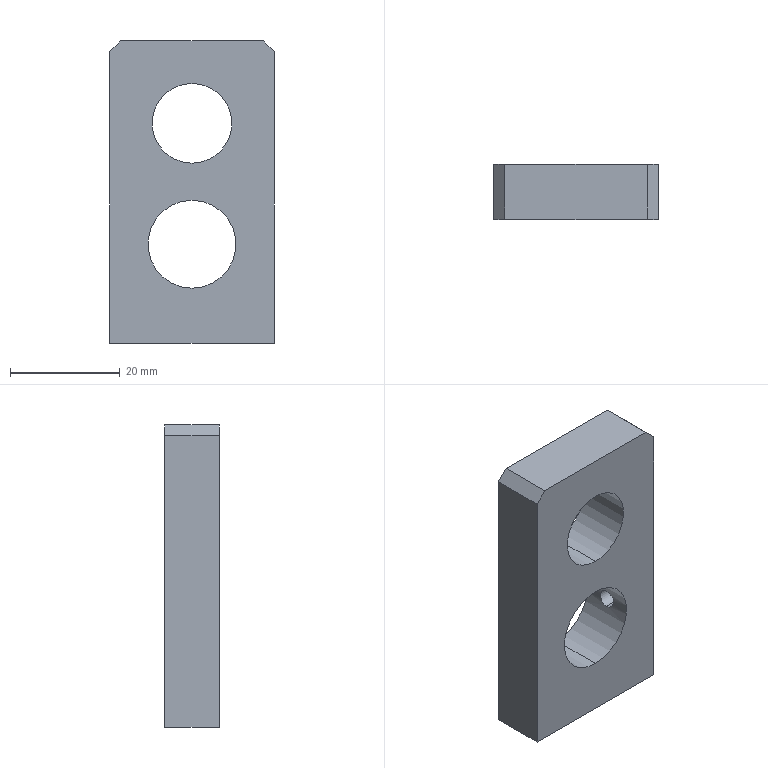Component | SolidWorks | GbgbMagnetSleeveSeatF8-4 | 1 solid | 22 faces | box 30 x 10 x 55 mm | volume 12559 mm3 | cylinder 10 | plane 8 | cone 4 | commonest cylinder face diameters 3.3 x6 14.5 x2 16 x2
build123d program:
from build123d import *

# Parameters (mm, degrees)
SKETCH1_W              = 30
SKETCH1_H              = 55
BOSS_EXTRUDE1_DEPTH    = 5
SKETCH2_R              = 6
CUT_EXTRUDE1_DEPTH     = 33.882
M4_TAPPED_HOLE2_D      = 3.3
M4_TAPPED_HOLE2_DEPTH  = 10.1
M4_TAPPED_HOLE2_TIP    = 0.9914
SKETCH12_R             = 8
CUT_EXTRUDE2_DEPTH     = 12
M16X1_5_TAPPED_HOLE1_D = 14.5
M4_TAPPED_HOLE3_D      = 3.3
M4_TAPPED_HOLE3_DEPTH  = 10.1
M4_TAPPED_HOLE3_TIP    = 0.9914
CHAMFER1_SIZE          = 2


with BuildPart() as part:
    # Sketch1 → Boss-Extrude1 (new, symmetric)
    with BuildSketch(Plane(origin=(0, 0, 0), x_dir=(1, 0, 0), z_dir=(0, 1, 0))):
        Rectangle(SKETCH1_W, SKETCH1_H)
    extrude(amount=BOSS_EXTRUDE1_DEPTH, both=True)

    # Sketch2 → Cut-Extrude1 (cut, through all)
    with BuildSketch(Plane(origin=(0, 5, 0), x_dir=(1, 0, 0), z_dir=(0, 1, 0))):
        with Locations(Location((0, -12.5, 0), (0, 0, 270))):
            Circle(SKETCH2_R)
    extrude(amount=-CUT_EXTRUDE1_DEPTH, mode=Mode.SUBTRACT)

    # M4 Tapped Hole2
    with Locations(Plane(origin=(2.316, -9.359, -27.5), x_dir=(1, 0, 0), z_dir=(0, 0, -1))):
        with Locations((7.684, -9.359), (-12.316, -9.359)):
            Hole(M4_TAPPED_HOLE2_D / 2, depth=M4_TAPPED_HOLE2_DEPTH)
            with Locations((0, 0, -(M4_TAPPED_HOLE2_DEPTH + M4_TAPPED_HOLE2_TIP / 2))):  # 118° drill point
                Cone(0, M4_TAPPED_HOLE2_D / 2, M4_TAPPED_HOLE2_TIP, mode=Mode.SUBTRACT)

    # Sketch12 → Cut-Extrude2 (cut)
    with BuildSketch(Plane(origin=(0, 5, 0), x_dir=(1, 0, 0), z_dir=(0, 1, 0))):
        with Locations(Location((0, 9.5, 0), (0, 0, 270))):
            Circle(SKETCH12_R)
    extrude(amount=-CUT_EXTRUDE2_DEPTH, mode=Mode.SUBTRACT)

    # M16x1.5 Tapped Hole1 (through all)
    with Locations(Plane(origin=(0, 5, 0), x_dir=(1, 0, 0), z_dir=(0, 1, 0))):
        with Locations((0, -12.5)):
            Hole(M16X1_5_TAPPED_HOLE1_D / 2)

    # M4 Tapped Hole3
    with Locations(Plane(origin=(15, 0, 0), x_dir=(0, 0, -1), z_dir=(1, 0, 0))):
        with Locations((9.5, 0)):
            Hole(M4_TAPPED_HOLE3_D / 2, depth=M4_TAPPED_HOLE3_DEPTH)
            with Locations((0, 0, -(M4_TAPPED_HOLE3_DEPTH + M4_TAPPED_HOLE3_TIP / 2))):  # 118° drill point
                Cone(0, M4_TAPPED_HOLE3_D / 2, M4_TAPPED_HOLE3_TIP, mode=Mode.SUBTRACT)

    # Chamfer1
    chamfer1_edges = [part.edges().sort_by_distance(p)[0] for p in [
        (15, 0, 27.5),
        (-15, 0, 27.5),
    ]]
    chamfer(chamfer1_edges, length=CHAMFER1_SIZE)


solid = part.part

# Placed as in the assembly
solid = solid.moved(Location((80.446, 494.94, 417.732), (0, 0, 0)))
STEP:
#1=CARTESIAN_POINT('',(3.475,19.486,16.137));
#2=VERTEX_POINT('',#1);
#3=CARTESIAN_POINT('',(3.475,19.486,16.007));
#4=VERTEX_POINT('',#3);
#5=CARTESIAN_POINT('',(3.475,19.486,16.137));
#6=CARTESIAN_POINT('',(3.475,19.477,16.137));
#7=CARTESIAN_POINT('',(3.476,19.469,16.135));
#8=CARTESIAN_POINT('',(3.477,19.457,16.13));
#9=CARTESIAN_POINT('',(3.477,19.453,16.128));
#10=CARTESIAN_POINT('',(3.478,19.446,16.124));
#11=CARTESIAN_POINT('',(3.478,19.443,16.121));
#12=CARTESIAN_POINT('',(3.479,19.437,16.115));
#13=CARTESIAN_POINT('',(3.48,19.434,16.112));
#14=CARTESIAN_POINT('',(3.48,19.429,16.105));
#15=CARTESIAN_POINT('',(3.481,19.427,16.101));
#16=CARTESIAN_POINT('',(3.482,19.423,16.089));
#17=CARTESIAN_POINT('',(3.482,19.421,16.081));
#18=CARTESIAN_POINT('',(3.482,19.421,16.068));
#19=CARTESIAN_POINT('',(3.482,19.421,16.064));
#20=CARTESIAN_POINT('',(3.482,19.423,16.055));
#21=CARTESIAN_POINT('',(3.481,19.424,16.051));
#22=CARTESIAN_POINT('',(3.481,19.427,16.043));
#23=CARTESIAN_POINT('',(3.48,19.429,16.04));
#24=CARTESIAN_POINT('',(3.48,19.434,16.033));
#25=CARTESIAN_POINT('',(3.479,19.437,16.029));
#26=CARTESIAN_POINT('',(3.478,19.446,16.02));
#27=CARTESIAN_POINT('',(3.477,19.453,16.015));
#28=CARTESIAN_POINT('',(3.476,19.465,16.011));
#29=CARTESIAN_POINT('',(3.476,19.469,16.009));
#30=CARTESIAN_POINT('',(3.475,19.477,16.008));
#31=CARTESIAN_POINT('',(3.475,19.482,16.007));
#32=CARTESIAN_POINT('',(3.475,19.486,16.007));
#33=B_SPLINE_CURVE_WITH_KNOTS('',3,(#5,#6,#7,#8,#9,#10,#11,#12,#13,#14,#15,#16,#17,#18,#19,#20,#21,#22,#23,#24,#25,#26,#27,#28,#29,#30,#31,#32),.UNSPECIFIED.,.F.,.F.,(4,2,2,2,2,2,2,2,2,2,2,2,2,4),(0.005173,0.005819,0.006142,0.006465,0.006789,0.007112,0.007758,0.008081,0.008405,0.008728,0.009051,0.009697,0.01002,0.01034),.UNSPECIFIED.);
#34=EDGE_CURVE('',#2,#4,#33,.T.);
#35=ORIENTED_EDGE('',*,*,#34,.F.);
#36=CARTESIAN_POINT('',(3.758,19.486,16.137));
#37=VERTEX_POINT('',#36);
#38=CARTESIAN_POINT('',(3.758,19.486,16.137));
#39=DIRECTION('',(1.,0.,-0.));
#40=VECTOR('',#39,39.37);
#41=LINE('',#38,#40);
#42=EDGE_CURVE('',#2,#37,#41,.T.);
#43=ORIENTED_EDGE('',*,*,#42,.T.);
#44=CARTESIAN_POINT('',(3.758,19.486,16.007));
#45=VERTEX_POINT('',#44);
#46=CARTESIAN_POINT('',(3.758,19.486,16.072));
#47=DIRECTION('',(1.,0.,-0.));
#48=DIRECTION('',(0.,0.,-1.));
#49=AXIS2_PLACEMENT_3D('',#46,#47,#48);
#50=CIRCLE('',#49,0.06496);
#51=EDGE_CURVE('',#37,#45,#50,.T.);
#52=ORIENTED_EDGE('',*,*,#51,.T.);
#53=CARTESIAN_POINT('',(3.758,19.486,16.007));
#54=DIRECTION('',(1.,0.,-0.));
#55=VECTOR('',#54,39.37);
#56=LINE('',#53,#55);
#57=EDGE_CURVE('',#4,#45,#56,.T.);
#58=ORIENTED_EDGE('',*,*,#57,.F.);
#59=EDGE_LOOP('',(#35,#43,#52,#58));
#60=FACE_OUTER_BOUND('',#59,.T.);
#61=CARTESIAN_POINT('',(3.758,19.486,16.072));
#62=DIRECTION('',(1.,0.,-0.));
#63=DIRECTION('',(0.,0.,-1.));
#64=AXIS2_PLACEMENT_3D('',#61,#62,#63);
#65=CYLINDRICAL_SURFACE('',#64,0.06496);
#66=ADVANCED_FACE('',(#60),#65,.F.);
#67=CARTESIAN_POINT('',(3.167,19.289,16.653));
#68=VERTEX_POINT('',#67);
#69=CARTESIAN_POINT('',(3.167,19.289,17.224));
#70=VERTEX_POINT('',#69);
#71=CARTESIAN_POINT('',(3.167,19.289,16.938));
#72=DIRECTION('',(0.,1.,0.));
#73=DIRECTION('',(0.,0.,1.));
#74=AXIS2_PLACEMENT_3D('',#71,#72,#73);
#75=CIRCLE('',#74,0.2854);
#76=EDGE_CURVE('',#68,#70,#75,.T.);
#77=ORIENTED_EDGE('',*,*,#76,.F.);
#78=CARTESIAN_POINT('',(3.167,19.683,16.653));
#79=VERTEX_POINT('',#78);
#80=CARTESIAN_POINT('',(3.167,19.683,16.653));
#81=DIRECTION('',(0.,1.,0.));
#82=VECTOR('',#81,39.37);
#83=LINE('',#80,#82);
#84=EDGE_CURVE('',#68,#79,#83,.T.);
#85=ORIENTED_EDGE('',*,*,#84,.T.);
#86=CARTESIAN_POINT('',(3.167,19.683,17.224));
#87=VERTEX_POINT('',#86);
#88=CARTESIAN_POINT('',(3.167,19.683,16.938));
#89=DIRECTION('',(0.,1.,0.));
#90=DIRECTION('',(0.,0.,1.));
#91=AXIS2_PLACEMENT_3D('',#88,#89,#90);
#92=CIRCLE('',#91,0.2854);
#93=EDGE_CURVE('',#79,#87,#92,.T.);
#94=ORIENTED_EDGE('',*,*,#93,.T.);
#95=CARTESIAN_POINT('',(3.167,19.683,17.224));
#96=DIRECTION('',(0.,1.,0.));
#97=VECTOR('',#96,39.37);
#98=LINE('',#95,#97);
#99=EDGE_CURVE('',#70,#87,#98,.T.);
#100=ORIENTED_EDGE('',*,*,#99,.F.);
#101=EDGE_LOOP('',(#77,#85,#94,#100));
#102=FACE_OUTER_BOUND('',#101,.T.);
#103=CARTESIAN_POINT('',(3.167,19.683,16.938));
#104=DIRECTION('',(0.,1.,0.));
#105=DIRECTION('',(0.,0.,1.));
#106=AXIS2_PLACEMENT_3D('',#103,#104,#105);
#107=CYLINDRICAL_SURFACE('',#106,0.2854);
#108=ADVANCED_FACE('',(#102),#107,.F.);
#109=CARTESIAN_POINT('',(3.167,19.289,15.757));
#110=VERTEX_POINT('',#109);
#111=CARTESIAN_POINT('',(3.167,19.289,16.387));
#112=VERTEX_POINT('',#111);
#113=CARTESIAN_POINT('',(3.167,19.289,16.072));
#114=DIRECTION('',(0.,1.,0.));
#115=DIRECTION('',(0.,0.,1.));
#116=AXIS2_PLACEMENT_3D('',#113,#114,#115);
#117=CIRCLE('',#116,0.315);
#118=EDGE_CURVE('',#110,#112,#117,.T.);
#119=ORIENTED_EDGE('',*,*,#118,.F.);
#120=CARTESIAN_POINT('',(3.167,19.683,15.757));
#121=VERTEX_POINT('',#120);
#122=CARTESIAN_POINT('',(3.167,19.21,15.757));
#123=DIRECTION('',(0.,1.,0.));
#124=VECTOR('',#123,39.37);
#125=LINE('',#122,#124);
#126=EDGE_CURVE('',#110,#121,#125,.T.);
#127=ORIENTED_EDGE('',*,*,#126,.T.);
#128=CARTESIAN_POINT('',(3.167,19.683,16.387));
#129=VERTEX_POINT('',#128);
#130=CARTESIAN_POINT('',(3.167,19.683,16.072));
#131=DIRECTION('',(0.,1.,0.));
#132=DIRECTION('',(0.,0.,1.));
#133=AXIS2_PLACEMENT_3D('',#130,#131,#132);
#134=CIRCLE('',#133,0.315);
#135=EDGE_CURVE('',#121,#129,#134,.T.);
#136=ORIENTED_EDGE('',*,*,#135,.T.);
#137=CARTESIAN_POINT('',(3.167,19.21,16.387));
#138=DIRECTION('',(0.,1.,0.));
#139=VECTOR('',#138,39.37);
#140=LINE('',#137,#139);
#141=EDGE_CURVE('',#112,#129,#140,.T.);
#142=ORIENTED_EDGE('',*,*,#141,.F.);
#143=EDGE_LOOP('',(#119,#127,#136,#142));
#144=FACE_OUTER_BOUND('',#143,.T.);
#145=CARTESIAN_POINT('',(3.167,19.21,16.072));
#146=DIRECTION('',(0.,1.,0.));
#147=DIRECTION('',(0.,0.,1.));
#148=AXIS2_PLACEMENT_3D('',#145,#146,#147);
#149=CYLINDRICAL_SURFACE('',#148,0.315);
#150=ADVANCED_FACE('',(#144),#149,.F.);
#151=CARTESIAN_POINT('',(3.626,19.486,15.761));
#152=VERTEX_POINT('',#151);
#153=CARTESIAN_POINT('',(3.496,19.486,15.761));
#154=VERTEX_POINT('',#153);
#155=CARTESIAN_POINT('',(3.561,19.486,15.761));
#156=DIRECTION('',(0.,0.,-1.));
#157=DIRECTION('',(-1.,0.,0.));
#158=AXIS2_PLACEMENT_3D('',#155,#156,#157);
#159=CIRCLE('',#158,0.06496);
#160=EDGE_CURVE('',#152,#154,#159,.T.);
#161=ORIENTED_EDGE('',*,*,#160,.F.);
#162=CARTESIAN_POINT('',(3.626,19.486,15.363));
#163=VERTEX_POINT('',#162);
#164=CARTESIAN_POINT('',(3.626,19.486,15.363));
#165=DIRECTION('',(0.,0.,-1.));
#166=VECTOR('',#165,39.37);
#167=LINE('',#164,#166);
#168=EDGE_CURVE('',#152,#163,#167,.T.);
#169=ORIENTED_EDGE('',*,*,#168,.T.);
#170=CARTESIAN_POINT('',(3.496,19.486,15.363));
#171=VERTEX_POINT('',#170);
#172=CARTESIAN_POINT('',(3.561,19.486,15.363));
#173=DIRECTION('',(0.,0.,-1.));
#174=DIRECTION('',(-1.,0.,0.));
#175=AXIS2_PLACEMENT_3D('',#172,#173,#174);
#176=CIRCLE('',#175,0.06496);
#177=EDGE_CURVE('',#163,#171,#176,.T.);
#178=ORIENTED_EDGE('',*,*,#177,.T.);
#179=CARTESIAN_POINT('',(3.496,19.486,15.363));
#180=DIRECTION('',(0.,0.,-1.));
#181=VECTOR('',#180,39.37);
#182=LINE('',#179,#181);
#183=EDGE_CURVE('',#154,#171,#182,.T.);
#184=ORIENTED_EDGE('',*,*,#183,.F.);
#185=EDGE_LOOP('',(#161,#169,#178,#184));
#186=FACE_OUTER_BOUND('',#185,.T.);
#187=CARTESIAN_POINT('',(3.561,19.486,15.363));
#188=DIRECTION('',(0.,0.,-1.));
#189=DIRECTION('',(-1.,0.,0.));
#190=AXIS2_PLACEMENT_3D('',#187,#188,#189);
#191=CYLINDRICAL_SURFACE('',#190,0.06496);
#192=ADVANCED_FACE('',(#186),#191,.F.);
#193=CARTESIAN_POINT('',(3.561,19.486,15.8));
#194=VERTEX_POINT('',#193);
#195=CARTESIAN_POINT('',(3.496,19.486,15.761));
#196=DIRECTION('',(-0.8572,0.,-0.515));
#197=VECTOR('',#196,39.37);
#198=LINE('',#195,#197);
#199=EDGE_CURVE('',#194,#154,#198,.T.);
#200=ORIENTED_EDGE('',*,*,#199,.F.);
#201=CARTESIAN_POINT('',(3.626,19.486,15.761));
#202=DIRECTION('',(0.8572,0.,-0.515));
#203=VECTOR('',#202,39.37);
#204=LINE('',#201,#203);
#205=EDGE_CURVE('',#194,#152,#204,.T.);
#206=ORIENTED_EDGE('',*,*,#205,.T.);
#207=ORIENTED_EDGE('',*,*,#160,.T.);
#208=EDGE_LOOP('',(#200,#206,#207));
#209=FACE_OUTER_BOUND('',#208,.T.);
#210=CARTESIAN_POINT('',(3.561,19.486,15.761));
#211=DIRECTION('',(0.,0.,-1.));
#212=DIRECTION('',(-1.,0.,0.));
#213=AXIS2_PLACEMENT_3D('',#210,#211,#212);
#214=CONICAL_SURFACE('',#213,0.06496,1.03);
#215=ADVANCED_FACE('',(#209),#214,.F.);
#216=CARTESIAN_POINT('',(2.838,19.486,15.761));
#217=VERTEX_POINT('',#216);
#218=CARTESIAN_POINT('',(2.709,19.486,15.761));
#219=VERTEX_POINT('',#218);
#220=CARTESIAN_POINT('',(2.773,19.486,15.761));
#221=DIRECTION('',(0.,0.,-1.));
#222=DIRECTION('',(-1.,0.,0.));
#223=AXIS2_PLACEMENT_3D('',#220,#221,#222);
#224=CIRCLE('',#223,0.06496);
#225=EDGE_CURVE('',#217,#219,#224,.T.);
#226=ORIENTED_EDGE('',*,*,#225,.F.);
#227=CARTESIAN_POINT('',(2.838,19.486,15.363));
#228=VERTEX_POINT('',#227);
#229=CARTESIAN_POINT('',(2.838,19.486,15.363));
#230=DIRECTION('',(0.,0.,-1.));
#231=VECTOR('',#230,39.37);
#232=LINE('',#229,#231);
#233=EDGE_CURVE('',#217,#228,#232,.T.);
#234=ORIENTED_EDGE('',*,*,#233,.T.);
#235=CARTESIAN_POINT('',(2.709,19.486,15.363));
#236=VERTEX_POINT('',#235);
#237=CARTESIAN_POINT('',(2.773,19.486,15.363));
#238=DIRECTION('',(0.,0.,-1.));
#239=DIRECTION('',(-1.,0.,0.));
#240=AXIS2_PLACEMENT_3D('',#237,#238,#239);
#241=CIRCLE('',#240,0.06496);
#242=EDGE_CURVE('',#228,#236,#241,.T.);
#243=ORIENTED_EDGE('',*,*,#242,.T.);
#244=CARTESIAN_POINT('',(2.709,19.486,15.363));
#245=DIRECTION('',(0.,0.,-1.));
#246=VECTOR('',#245,39.37);
#247=LINE('',#244,#246);
#248=EDGE_CURVE('',#219,#236,#247,.T.);
#249=ORIENTED_EDGE('',*,*,#248,.F.);
#250=EDGE_LOOP('',(#226,#234,#243,#249));
#251=FACE_OUTER_BOUND('',#250,.T.);
#252=CARTESIAN_POINT('',(2.773,19.486,15.363));
#253=DIRECTION('',(0.,0.,-1.));
#254=DIRECTION('',(-1.,0.,0.));
#255=AXIS2_PLACEMENT_3D('',#252,#253,#254);
#256=CYLINDRICAL_SURFACE('',#255,0.06496);
#257=ADVANCED_FACE('',(#251),#256,.F.);
#258=CARTESIAN_POINT('',(2.773,19.486,15.8));
#259=VERTEX_POINT('',#258);
#260=CARTESIAN_POINT('',(2.709,19.486,15.761));
#261=DIRECTION('',(-0.8572,0.,-0.515));
#262=VECTOR('',#261,39.37);
#263=LINE('',#260,#262);
#264=EDGE_CURVE('',#259,#219,#263,.T.);
#265=ORIENTED_EDGE('',*,*,#264,.F.);
#266=CARTESIAN_POINT('',(2.838,19.486,15.761));
#267=DIRECTION('',(0.8572,0.,-0.515));
#268=VECTOR('',#267,39.37);
#269=LINE('',#266,#268);
#270=EDGE_CURVE('',#259,#217,#269,.T.);
#271=ORIENTED_EDGE('',*,*,#270,.T.);
#272=ORIENTED_EDGE('',*,*,#225,.T.);
#273=EDGE_LOOP('',(#265,#271,#272));
#274=FACE_OUTER_BOUND('',#273,.T.);
#275=CARTESIAN_POINT('',(2.773,19.486,15.761));
#276=DIRECTION('',(0.,0.,-1.));
#277=DIRECTION('',(-1.,0.,0.));
#278=AXIS2_PLACEMENT_3D('',#275,#276,#277);
#279=CONICAL_SURFACE('',#278,0.06496,1.03);
#280=ADVANCED_FACE('',(#274),#279,.F.);
#281=CARTESIAN_POINT('',(3.758,19.486,16.072));
#282=DIRECTION('',(1.,0.,-0.));
#283=DIRECTION('',(0.,0.,-1.));
#284=AXIS2_PLACEMENT_3D('',#281,#282,#283);
#285=CIRCLE('',#284,0.06496);
#286=EDGE_CURVE('',#45,#37,#285,.T.);
#287=ORIENTED_EDGE('',*,*,#286,.F.);
#288=ORIENTED_EDGE('',*,*,#51,.F.);
#289=EDGE_LOOP('',(#287,#288));
#290=FACE_BOUND('',#289,.T.);
#291=CARTESIAN_POINT('',(3.758,19.683,17.45));
#292=VERTEX_POINT('',#291);
#293=CARTESIAN_POINT('',(3.758,19.683,15.363));
#294=VERTEX_POINT('',#293);
#295=CARTESIAN_POINT('',(3.758,19.683,15.363));
#296=DIRECTION('',(-0.,0.,-1.));
#297=VECTOR('',#296,39.37);
#298=LINE('',#295,#297);
#299=EDGE_CURVE('',#292,#294,#298,.T.);
#300=ORIENTED_EDGE('',*,*,#299,.F.);
#301=CARTESIAN_POINT('',(3.758,19.289,17.45));
#302=VERTEX_POINT('',#301);
#303=CARTESIAN_POINT('',(3.758,19.683,17.45));
#304=DIRECTION('',(0.,-1.,0.));
#305=VECTOR('',#304,39.37);
#306=LINE('',#303,#305);
#307=EDGE_CURVE('',#292,#302,#306,.T.);
#308=ORIENTED_EDGE('',*,*,#307,.T.);
#309=CARTESIAN_POINT('',(3.758,19.289,15.363));
#310=VERTEX_POINT('',#309);
#311=CARTESIAN_POINT('',(3.758,19.289,15.363));
#312=DIRECTION('',(-0.,0.,-1.));
#313=VECTOR('',#312,39.37);
#314=LINE('',#311,#313);
#315=EDGE_CURVE('',#302,#310,#314,.T.);
#316=ORIENTED_EDGE('',*,*,#315,.T.);
#317=CARTESIAN_POINT('',(3.758,19.683,15.363));
#318=DIRECTION('',(0.,-1.,0.));
#319=VECTOR('',#318,39.37);
#320=LINE('',#317,#319);
#321=EDGE_CURVE('',#294,#310,#320,.T.);
#322=ORIENTED_EDGE('',*,*,#321,.F.);
#323=EDGE_LOOP('',(#300,#308,#316,#322));
#324=FACE_OUTER_BOUND('',#323,.T.);
#325=CARTESIAN_POINT('',(3.758,19.683,15.363));
#326=DIRECTION('',(-1.,0.,0.));
#327=DIRECTION('',(0.,0.,1.));
#328=AXIS2_PLACEMENT_3D('',#325,#326,#327);
#329=PLANE('',#328);
#330=ADVANCED_FACE('',(#290,#324),#329,.F.);
#331=CARTESIAN_POINT('',(3.561,19.486,15.363));
#332=DIRECTION('',(0.,0.,-1.));
#333=DIRECTION('',(-1.,0.,0.));
#334=AXIS2_PLACEMENT_3D('',#331,#332,#333);
#335=CIRCLE('',#334,0.06496);
#336=EDGE_CURVE('',#171,#163,#335,.T.);
#337=ORIENTED_EDGE('',*,*,#336,.F.);
#338=ORIENTED_EDGE('',*,*,#177,.F.);
#339=EDGE_LOOP('',(#337,#338));
#340=FACE_BOUND('',#339,.T.);
#341=CARTESIAN_POINT('',(2.773,19.486,15.363));
#342=DIRECTION('',(0.,0.,-1.));
#343=DIRECTION('',(-1.,0.,0.));
#344=AXIS2_PLACEMENT_3D('',#341,#342,#343);
#345=CIRCLE('',#344,0.06496);
#346=EDGE_CURVE('',#236,#228,#345,.T.);
#347=ORIENTED_EDGE('',*,*,#346,.F.);
#348=ORIENTED_EDGE('',*,*,#242,.F.);
#349=EDGE_LOOP('',(#347,#348));
#350=FACE_BOUND('',#349,.T.);
#351=CARTESIAN_POINT('',(2.577,19.289,15.363));
#352=VERTEX_POINT('',#351);
#353=CARTESIAN_POINT('',(2.577,19.289,15.363));
#354=DIRECTION('',(-1.,0.,0.));
#355=VECTOR('',#354,39.37);
#356=LINE('',#353,#355);
#357=EDGE_CURVE('',#310,#352,#356,.T.);
#358=ORIENTED_EDGE('',*,*,#357,.T.);
#359=CARTESIAN_POINT('',(2.577,19.683,15.363));
#360=VERTEX_POINT('',#359);
#361=CARTESIAN_POINT('',(2.577,19.683,15.363));
#362=DIRECTION('',(0.,-1.,0.));
#363=VECTOR('',#362,39.37);
#364=LINE('',#361,#363);
#365=EDGE_CURVE('',#360,#352,#364,.T.);
#366=ORIENTED_EDGE('',*,*,#365,.F.);
#367=CARTESIAN_POINT('',(2.577,19.683,15.363));
#368=DIRECTION('',(-1.,0.,0.));
#369=VECTOR('',#368,39.37);
#370=LINE('',#367,#369);
#371=EDGE_CURVE('',#294,#360,#370,.T.);
#372=ORIENTED_EDGE('',*,*,#371,.F.);
#373=ORIENTED_EDGE('',*,*,#321,.T.);
#374=EDGE_LOOP('',(#358,#366,#372,#373));
#375=FACE_OUTER_BOUND('',#374,.T.);
#376=CARTESIAN_POINT('',(2.577,19.683,15.363));
#377=DIRECTION('',(0.,0.,1.));
#378=DIRECTION('',(1.,0.,0.));
#379=AXIS2_PLACEMENT_3D('',#376,#377,#378);
#380=PLANE('',#379);
#381=ADVANCED_FACE('',(#340,#350,#375),#380,.F.);
#382=CARTESIAN_POINT('',(2.577,19.289,17.45));
#383=VERTEX_POINT('',#382);
#384=CARTESIAN_POINT('',(2.577,19.289,15.363));
#385=DIRECTION('',(0.,0.,1.));
#386=VECTOR('',#385,39.37);
#387=LINE('',#384,#386);
#388=EDGE_CURVE('',#352,#383,#387,.T.);
#389=ORIENTED_EDGE('',*,*,#388,.T.);
#390=CARTESIAN_POINT('',(2.577,19.683,17.45));
#391=VERTEX_POINT('',#390);
#392=CARTESIAN_POINT('',(2.577,19.683,17.45));
#393=DIRECTION('',(0.,1.,0.));
#394=VECTOR('',#393,39.37);
#395=LINE('',#392,#394);
#396=EDGE_CURVE('',#383,#391,#395,.T.);
#397=ORIENTED_EDGE('',*,*,#396,.T.);
#398=CARTESIAN_POINT('',(2.577,19.683,15.363));
#399=DIRECTION('',(0.,0.,1.));
#400=VECTOR('',#399,39.37);
#401=LINE('',#398,#400);
#402=EDGE_CURVE('',#360,#391,#401,.T.);
#403=ORIENTED_EDGE('',*,*,#402,.F.);
#404=ORIENTED_EDGE('',*,*,#365,.T.);
#405=EDGE_LOOP('',(#389,#397,#403,#404));
#406=FACE_OUTER_BOUND('',#405,.T.);
#407=CARTESIAN_POINT('',(2.577,19.683,15.363));
#408=DIRECTION('',(1.,0.,-0.));
#409=DIRECTION('',(-0.,0.,-1.));
#410=AXIS2_PLACEMENT_3D('',#407,#408,#409);
#411=PLANE('',#410);
#412=ADVANCED_FACE('',(#406),#411,.F.);
#413=CARTESIAN_POINT('',(2.655,19.289,17.529));
#414=VERTEX_POINT('',#413);
#415=CARTESIAN_POINT('',(3.679,19.289,17.529));
#416=VERTEX_POINT('',#415);
#417=CARTESIAN_POINT('',(2.577,19.289,17.529));
#418=DIRECTION('',(1.,0.,0.));
#419=VECTOR('',#418,39.37);
#420=LINE('',#417,#419);
#421=EDGE_CURVE('',#414,#416,#420,.T.);
#422=ORIENTED_EDGE('',*,*,#421,.T.);
#423=CARTESIAN_POINT('',(3.679,19.683,17.529));
#424=VERTEX_POINT('',#423);
#425=CARTESIAN_POINT('',(3.679,19.683,17.529));
#426=DIRECTION('',(0.,1.,0.));
#427=VECTOR('',#426,39.37);
#428=LINE('',#425,#427);
#429=EDGE_CURVE('',#416,#424,#428,.T.);
#430=ORIENTED_EDGE('',*,*,#429,.T.);
#431=CARTESIAN_POINT('',(2.655,19.683,17.529));
#432=VERTEX_POINT('',#431);
#433=CARTESIAN_POINT('',(2.577,19.683,17.529));
#434=DIRECTION('',(1.,0.,0.));
#435=VECTOR('',#434,39.37);
#436=LINE('',#433,#435);
#437=EDGE_CURVE('',#432,#424,#436,.T.);
#438=ORIENTED_EDGE('',*,*,#437,.F.);
#439=CARTESIAN_POINT('',(2.655,19.683,17.529));
#440=DIRECTION('',(0.,-1.,0.));
#441=VECTOR('',#440,39.37);
#442=LINE('',#439,#441);
#443=EDGE_CURVE('',#432,#414,#442,.T.);
#444=ORIENTED_EDGE('',*,*,#443,.T.);
#445=EDGE_LOOP('',(#422,#430,#438,#444));
#446=FACE_OUTER_BOUND('',#445,.T.);
#447=CARTESIAN_POINT('',(2.577,19.683,17.529));
#448=DIRECTION('',(0.,0.,-1.));
#449=DIRECTION('',(-1.,0.,0.));
#450=AXIS2_PLACEMENT_3D('',#447,#448,#449);
#451=PLANE('',#450);
#452=ADVANCED_FACE('',(#446),#451,.F.);
#453=CARTESIAN_POINT('',(3.167,19.683,16.938));
#454=DIRECTION('',(0.,1.,0.));
#455=DIRECTION('',(0.,0.,1.));
#456=AXIS2_PLACEMENT_3D('',#453,#454,#455);
#457=CIRCLE('',#456,0.2854);
#458=EDGE_CURVE('',#87,#79,#457,.T.);
#459=ORIENTED_EDGE('',*,*,#458,.F.);
#460=ORIENTED_EDGE('',*,*,#93,.F.);
#461=EDGE_LOOP('',(#459,#460));
#462=FACE_BOUND('',#461,.T.);
#463=CARTESIAN_POINT('',(3.167,19.683,16.072));
#464=DIRECTION('',(0.,1.,0.));
#465=DIRECTION('',(0.,0.,1.));
#466=AXIS2_PLACEMENT_3D('',#463,#464,#465);
#467=CIRCLE('',#466,0.315);
#468=EDGE_CURVE('',#129,#121,#467,.T.);
#469=ORIENTED_EDGE('',*,*,#468,.F.);
#470=ORIENTED_EDGE('',*,*,#135,.F.);
#471=EDGE_LOOP('',(#469,#470));
#472=FACE_BOUND('',#471,.T.);
#473=ORIENTED_EDGE('',*,*,#437,.T.);
#474=CARTESIAN_POINT('',(3.964,19.683,17.243));
#475=DIRECTION('',(0.7071,0.,-0.7071));
#476=VECTOR('',#475,39.37);
#477=LINE('',#474,#476);
#478=EDGE_CURVE('',#424,#292,#477,.T.);
#479=ORIENTED_EDGE('',*,*,#478,.T.);
#480=ORIENTED_EDGE('',*,*,#299,.T.);
#481=ORIENTED_EDGE('',*,*,#371,.T.);
#482=ORIENTED_EDGE('',*,*,#402,.T.);
#483=CARTESIAN_POINT('',(2.37,19.683,17.243));
#484=DIRECTION('',(0.7071,0.,0.7071));
#485=VECTOR('',#484,39.37);
#486=LINE('',#483,#485);
#487=EDGE_CURVE('',#391,#432,#486,.T.);
#488=ORIENTED_EDGE('',*,*,#487,.T.);
#489=EDGE_LOOP('',(#473,#479,#480,#481,#482,#488));
#490=FACE_OUTER_BOUND('',#489,.T.);
#491=CARTESIAN_POINT('',(3.167,19.683,16.446));
#492=DIRECTION('',(0.,1.,0.));
#493=DIRECTION('',(0.,0.,1.));
#494=AXIS2_PLACEMENT_3D('',#491,#492,#493);
#495=PLANE('',#494);
#496=ADVANCED_FACE('',(#462,#472,#490),#495,.T.);
#497=CARTESIAN_POINT('',(3.167,19.289,16.938));
#498=DIRECTION('',(0.,1.,0.));
#499=DIRECTION('',(0.,0.,1.));
#500=AXIS2_PLACEMENT_3D('',#497,#498,#499);
#501=CIRCLE('',#500,0.2854);
#502=EDGE_CURVE('',#70,#68,#501,.T.);
#503=ORIENTED_EDGE('',*,*,#502,.T.);
#504=ORIENTED_EDGE('',*,*,#76,.T.);
#505=EDGE_LOOP('',(#503,#504));
#506=FACE_BOUND('',#505,.T.);
#507=CARTESIAN_POINT('',(3.167,19.289,16.072));
#508=DIRECTION('',(0.,1.,0.));
#509=DIRECTION('',(0.,0.,1.));
#510=AXIS2_PLACEMENT_3D('',#507,#508,#509);
#511=CIRCLE('',#510,0.315);
#512=EDGE_CURVE('',#112,#110,#511,.T.);
#513=ORIENTED_EDGE('',*,*,#512,.T.);
#514=ORIENTED_EDGE('',*,*,#118,.T.);
#515=EDGE_LOOP('',(#513,#514));
#516=FACE_BOUND('',#515,.T.);
#517=ORIENTED_EDGE('',*,*,#315,.F.);
#518=CARTESIAN_POINT('',(3.758,19.289,17.45));
#519=DIRECTION('',(-0.7071,0.,0.7071));
#520=VECTOR('',#519,39.37);
#521=LINE('',#518,#520);
#522=EDGE_CURVE('',#302,#416,#521,.T.);
#523=ORIENTED_EDGE('',*,*,#522,.T.);
#524=ORIENTED_EDGE('',*,*,#421,.F.);
#525=CARTESIAN_POINT('',(2.655,19.289,17.529));
#526=DIRECTION('',(-0.7071,0.,-0.7071));
#527=VECTOR('',#526,39.37);
#528=LINE('',#525,#527);
#529=EDGE_CURVE('',#414,#383,#528,.T.);
#530=ORIENTED_EDGE('',*,*,#529,.T.);
#531=ORIENTED_EDGE('',*,*,#388,.F.);
#532=ORIENTED_EDGE('',*,*,#357,.F.);
#533=EDGE_LOOP('',(#517,#523,#524,#530,#531,#532));
#534=FACE_OUTER_BOUND('',#533,.T.);
#535=CARTESIAN_POINT('',(3.167,19.289,16.446));
#536=DIRECTION('',(0.,1.,0.));
#537=DIRECTION('',(0.,0.,1.));
#538=AXIS2_PLACEMENT_3D('',#535,#536,#537);
#539=PLANE('',#538);
#540=ADVANCED_FACE('',(#506,#516,#534),#539,.F.);
#541=ORIENTED_EDGE('',*,*,#270,.F.);
#542=ORIENTED_EDGE('',*,*,#264,.T.);
#543=CARTESIAN_POINT('',(2.773,19.486,15.761));
#544=DIRECTION('',(0.,0.,-1.));
#545=DIRECTION('',(-1.,0.,0.));
#546=AXIS2_PLACEMENT_3D('',#543,#544,#545);
#547=CIRCLE('',#546,0.06496);
#548=EDGE_CURVE('',#219,#217,#547,.T.);
#549=ORIENTED_EDGE('',*,*,#548,.T.);
#550=EDGE_LOOP('',(#541,#542,#549));
#551=FACE_OUTER_BOUND('',#550,.T.);
#552=CARTESIAN_POINT('',(2.773,19.486,15.761));
#553=DIRECTION('',(0.,0.,-1.));
#554=DIRECTION('',(-1.,0.,0.));
#555=AXIS2_PLACEMENT_3D('',#552,#553,#554);
#556=CONICAL_SURFACE('',#555,0.06496,1.03);
#557=ADVANCED_FACE('',(#551),#556,.F.);
#558=ORIENTED_EDGE('',*,*,#233,.F.);
#559=ORIENTED_EDGE('',*,*,#548,.F.);
#560=ORIENTED_EDGE('',*,*,#248,.T.);
#561=ORIENTED_EDGE('',*,*,#346,.T.);
#562=EDGE_LOOP('',(#558,#559,#560,#561));
#563=FACE_OUTER_BOUND('',#562,.T.);
#564=CARTESIAN_POINT('',(2.773,19.486,15.363));
#565=DIRECTION('',(0.,0.,-1.));
#566=DIRECTION('',(-1.,0.,0.));
#567=AXIS2_PLACEMENT_3D('',#564,#565,#566);
#568=CYLINDRICAL_SURFACE('',#567,0.06496);
#569=ADVANCED_FACE('',(#563),#568,.F.);
#570=ORIENTED_EDGE('',*,*,#205,.F.);
#571=ORIENTED_EDGE('',*,*,#199,.T.);
#572=CARTESIAN_POINT('',(3.561,19.486,15.761));
#573=DIRECTION('',(0.,0.,-1.));
#574=DIRECTION('',(-1.,0.,0.));
#575=AXIS2_PLACEMENT_3D('',#572,#573,#574);
#576=CIRCLE('',#575,0.06496);
#577=EDGE_CURVE('',#154,#152,#576,.T.);
#578=ORIENTED_EDGE('',*,*,#577,.T.);
#579=EDGE_LOOP('',(#570,#571,#578));
#580=FACE_OUTER_BOUND('',#579,.T.);
#581=CARTESIAN_POINT('',(3.561,19.486,15.761));
#582=DIRECTION('',(0.,0.,-1.));
#583=DIRECTION('',(-1.,0.,0.));
#584=AXIS2_PLACEMENT_3D('',#581,#582,#583);
#585=CONICAL_SURFACE('',#584,0.06496,1.03);
#586=ADVANCED_FACE('',(#580),#585,.F.);
#587=ORIENTED_EDGE('',*,*,#168,.F.);
#588=ORIENTED_EDGE('',*,*,#577,.F.);
#589=ORIENTED_EDGE('',*,*,#183,.T.);
#590=ORIENTED_EDGE('',*,*,#336,.T.);
#591=EDGE_LOOP('',(#587,#588,#589,#590));
#592=FACE_OUTER_BOUND('',#591,.T.);
#593=CARTESIAN_POINT('',(3.561,19.486,15.363));
#594=DIRECTION('',(0.,0.,-1.));
#595=DIRECTION('',(-1.,0.,0.));
#596=AXIS2_PLACEMENT_3D('',#593,#594,#595);
#597=CYLINDRICAL_SURFACE('',#596,0.06496);
#598=ADVANCED_FACE('',(#592),#597,.F.);
#599=ORIENTED_EDGE('',*,*,#126,.F.);
#600=ORIENTED_EDGE('',*,*,#512,.F.);
#601=ORIENTED_EDGE('',*,*,#141,.T.);
#602=ORIENTED_EDGE('',*,*,#468,.T.);
#603=EDGE_LOOP('',(#599,#600,#601,#602));
#604=FACE_OUTER_BOUND('',#603,.T.);
#605=CARTESIAN_POINT('',(3.475,19.486,16.007));
#606=CARTESIAN_POINT('',(3.475,19.49,16.007));
#607=CARTESIAN_POINT('',(3.475,19.494,16.008));
#608=CARTESIAN_POINT('',(3.476,19.503,16.009));
#609=CARTESIAN_POINT('',(3.476,19.507,16.01));
#610=CARTESIAN_POINT('',(3.477,19.515,16.014));
#611=CARTESIAN_POINT('',(3.477,19.518,16.016));
#612=CARTESIAN_POINT('',(3.478,19.525,16.02));
#613=CARTESIAN_POINT('',(3.478,19.529,16.023));
#614=CARTESIAN_POINT('',(3.48,19.538,16.032));
#615=CARTESIAN_POINT('',(3.481,19.543,16.039));
#616=CARTESIAN_POINT('',(3.482,19.549,16.055));
#617=CARTESIAN_POINT('',(3.482,19.551,16.064));
#618=CARTESIAN_POINT('',(3.482,19.551,16.076));
#619=CARTESIAN_POINT('',(3.482,19.55,16.081));
#620=CARTESIAN_POINT('',(3.482,19.549,16.089));
#621=CARTESIAN_POINT('',(3.481,19.547,16.093));
#622=CARTESIAN_POINT('',(3.481,19.543,16.105));
#623=CARTESIAN_POINT('',(3.48,19.538,16.112));
#624=CARTESIAN_POINT('',(3.478,19.529,16.121));
#625=CARTESIAN_POINT('',(3.478,19.525,16.124));
#626=CARTESIAN_POINT('',(3.477,19.518,16.128));
#627=CARTESIAN_POINT('',(3.477,19.515,16.13));
#628=CARTESIAN_POINT('',(3.476,19.507,16.134));
#629=CARTESIAN_POINT('',(3.476,19.503,16.135));
#630=CARTESIAN_POINT('',(3.475,19.494,16.137));
#631=CARTESIAN_POINT('',(3.475,19.49,16.137));
#632=CARTESIAN_POINT('',(3.475,19.486,16.137));
#633=B_SPLINE_CURVE_WITH_KNOTS('',3,(#605,#606,#607,#608,#609,#610,#611,#612,#613,#614,#615,#616,#617,#618,#619,#620,#621,#622,#623,#624,#625,#626,#627,#628,#629,#630,#631,#632),.UNSPECIFIED.,.F.,.F.,(4,2,2,2,2,2,2,2,2,2,2,2,2,4),(0.,0.0003233,0.0006466,0.0009699,0.001293,0.00194,0.002586,0.00291,0.003233,0.003879,0.004203,0.004526,0.004849,0.005173),.UNSPECIFIED.);
#634=EDGE_CURVE('',#4,#2,#633,.T.);
#635=ORIENTED_EDGE('',*,*,#634,.T.);
#636=ORIENTED_EDGE('',*,*,#34,.T.);
#637=EDGE_LOOP('',(#635,#636));
#638=FACE_BOUND('',#637,.T.);
#639=CARTESIAN_POINT('',(3.167,19.21,16.072));
#640=DIRECTION('',(0.,1.,0.));
#641=DIRECTION('',(0.,0.,1.));
#642=AXIS2_PLACEMENT_3D('',#639,#640,#641);
#643=CYLINDRICAL_SURFACE('',#642,0.315);
#644=ADVANCED_FACE('',(#604,#638),#643,.F.);
#645=ORIENTED_EDGE('',*,*,#84,.F.);
#646=ORIENTED_EDGE('',*,*,#502,.F.);
#647=ORIENTED_EDGE('',*,*,#99,.T.);
#648=ORIENTED_EDGE('',*,*,#458,.T.);
#649=EDGE_LOOP('',(#645,#646,#647,#648));
#650=FACE_OUTER_BOUND('',#649,.T.);
#651=CARTESIAN_POINT('',(3.167,19.683,16.938));
#652=DIRECTION('',(0.,1.,0.));
#653=DIRECTION('',(0.,0.,1.));
#654=AXIS2_PLACEMENT_3D('',#651,#652,#653);
#655=CYLINDRICAL_SURFACE('',#654,0.2854);
#656=ADVANCED_FACE('',(#650),#655,.F.);
#657=ORIENTED_EDGE('',*,*,#42,.F.);
#658=ORIENTED_EDGE('',*,*,#634,.F.);
#659=ORIENTED_EDGE('',*,*,#57,.T.);
#660=ORIENTED_EDGE('',*,*,#286,.T.);
#661=EDGE_LOOP('',(#657,#658,#659,#660));
#662=FACE_OUTER_BOUND('',#661,.T.);
#663=CARTESIAN_POINT('',(3.758,19.486,16.072));
#664=DIRECTION('',(1.,0.,-0.));
#665=DIRECTION('',(0.,0.,-1.));
#666=AXIS2_PLACEMENT_3D('',#663,#664,#665);
#667=CYLINDRICAL_SURFACE('',#666,0.06496);
#668=ADVANCED_FACE('',(#662),#667,.F.);
#669=ORIENTED_EDGE('',*,*,#478,.F.);
#670=ORIENTED_EDGE('',*,*,#429,.F.);
#671=ORIENTED_EDGE('',*,*,#522,.F.);
#672=ORIENTED_EDGE('',*,*,#307,.F.);
#673=EDGE_LOOP('',(#669,#670,#671,#672));
#674=FACE_OUTER_BOUND('',#673,.T.);
#675=CARTESIAN_POINT('',(3.758,19.683,17.45));
#676=DIRECTION('',(-0.7071,0.,-0.7071));
#677=DIRECTION('',(0.,-1.,0.));
#678=AXIS2_PLACEMENT_3D('',#675,#676,#677);
#679=PLANE('',#678);
#680=ADVANCED_FACE('',(#674),#679,.F.);
#681=ORIENTED_EDGE('',*,*,#487,.F.);
#682=ORIENTED_EDGE('',*,*,#396,.F.);
#683=ORIENTED_EDGE('',*,*,#529,.F.);
#684=ORIENTED_EDGE('',*,*,#443,.F.);
#685=EDGE_LOOP('',(#681,#682,#683,#684));
#686=FACE_OUTER_BOUND('',#685,.T.);
#687=CARTESIAN_POINT('',(2.655,19.683,17.529));
#688=DIRECTION('',(0.7071,0.,-0.7071));
#689=DIRECTION('',(0.,-1.,0.));
#690=AXIS2_PLACEMENT_3D('',#687,#688,#689);
#691=PLANE('',#690);
#692=ADVANCED_FACE('',(#686),#691,.F.);
#693=CLOSED_SHELL('',(#66,#108,#150,#192,#215,#257,#280,#330,#381,#412,#452,#496,#540,#557,#569,#586,#598,#644,#656,#668,#680,#692));
#694=MANIFOLD_SOLID_BREP('',#693);
#695=CARTESIAN_POINT('',(0.,0.,0.));
#696=DIRECTION('',(0.,0.,1.));
#697=DIRECTION('',(1.,0.,0.));
#698=AXIS2_PLACEMENT_3D('',#695,#696,#697);
#699=(LENGTH_UNIT()NAMED_UNIT(*)SI_UNIT($,.METRE.));
#700=LENGTH_MEASURE_WITH_UNIT(LENGTH_MEASURE(0.0254),#699);
#701=DIMENSIONAL_EXPONENTS(1.,0.,0.,0.,0.,0.,0.);
#702=(CONVERSION_BASED_UNIT('',#700)LENGTH_UNIT()NAMED_UNIT(#701));
#703=UNCERTAINTY_MEASURE_WITH_UNIT(LENGTH_MEASURE(0.00001),#702,'','');
#704=(NAMED_UNIT(*)PLANE_ANGLE_UNIT()SI_UNIT($,.RADIAN.));
#705=(NAMED_UNIT(*)SI_UNIT($,.STERADIAN.)SOLID_ANGLE_UNIT());
#706=(GEOMETRIC_REPRESENTATION_CONTEXT(3)GLOBAL_UNCERTAINTY_ASSIGNED_CONTEXT((#703))GLOBAL_UNIT_ASSIGNED_CONTEXT((#702,#704,#705))REPRESENTATION_CONTEXT('',''));
#707=ADVANCED_BREP_SHAPE_REPRESENTATION('',(#694,#698),#706);
#708=COLOUR_RGB('',0.7922,0.8196,0.9333);
#709=FILL_AREA_STYLE_COLOUR('',#708);
#710=FILL_AREA_STYLE('',(#709));
#711=SURFACE_STYLE_FILL_AREA(#710);
#712=SURFACE_SIDE_STYLE('',(#711));
#713=SURFACE_STYLE_USAGE(.BOTH.,#712);
#714=PRESENTATION_STYLE_ASSIGNMENT((#713));
#715=STYLED_ITEM('',(#714),#694);
#716=PRESENTATION_LAYER_ASSIGNMENT('','',(#715));
#717=(LENGTH_UNIT()NAMED_UNIT(*)SI_UNIT($,.METRE.));
#718=LENGTH_MEASURE_WITH_UNIT(LENGTH_MEASURE(0.0254),#717);
#719=DIMENSIONAL_EXPONENTS(1.,0.,0.,0.,0.,0.,0.);
#720=(CONVERSION_BASED_UNIT('',#718)LENGTH_UNIT()NAMED_UNIT(#719));
#721=UNCERTAINTY_MEASURE_WITH_UNIT(LENGTH_MEASURE(0.00001),#720,'','');
#722=(NAMED_UNIT(*)PLANE_ANGLE_UNIT()SI_UNIT($,.RADIAN.));
#723=(NAMED_UNIT(*)SI_UNIT($,.STERADIAN.)SOLID_ANGLE_UNIT());
#724=(GEOMETRIC_REPRESENTATION_CONTEXT(3)GLOBAL_UNCERTAINTY_ASSIGNED_CONTEXT((#721))GLOBAL_UNIT_ASSIGNED_CONTEXT((#720,#722,#723))REPRESENTATION_CONTEXT('',''));
#725=MECHANICAL_DESIGN_GEOMETRIC_PRESENTATION_REPRESENTATION('',(#715),#724);